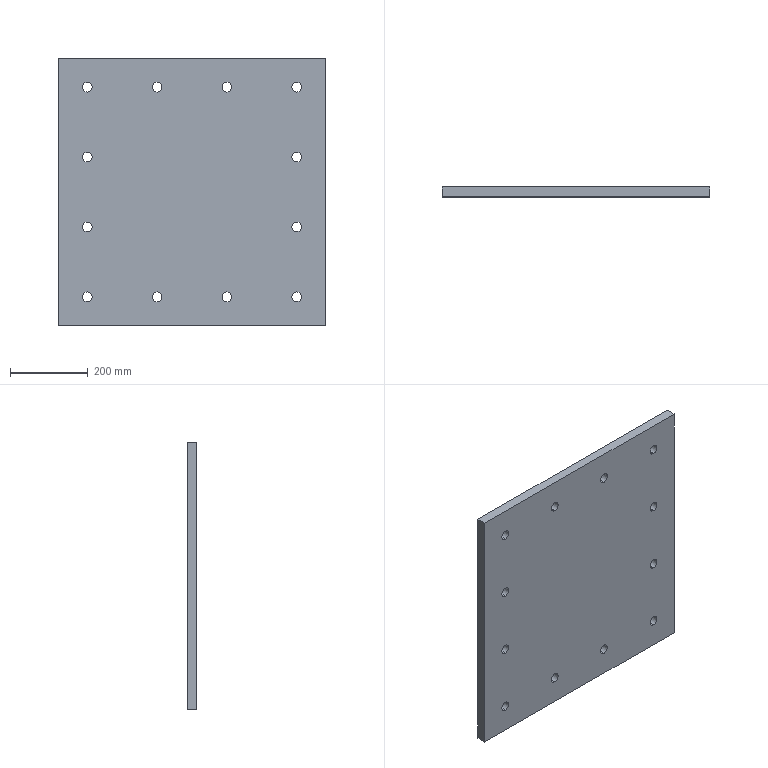Component | SolidWorks | Flange25-5 | 1 solid | 30 faces | box 690 x 25 x 690 mm | volume 11755238 mm3 | cylinder 24 | plane 6 | commonest cylinder face diameters 25 x24 | material Plain Carbon Steel
STEP:
#1=COLOUR_RGB('',0.7922,0.8196,0.9333);
#2=FILL_AREA_STYLE_COLOUR('',#1);
#3=FILL_AREA_STYLE('',(#2));
#4=SURFACE_STYLE_FILL_AREA(#3);
#5=SURFACE_SIDE_STYLE('',(#4));
#6=SURFACE_STYLE_USAGE(.BOTH.,#5);
#7=PRESENTATION_STYLE_ASSIGNMENT((#6));
#8=CARTESIAN_POINT('',(674.21,46.055,62.905));
#9=VERTEX_POINT('',#8);
#10=CARTESIAN_POINT('',(674.21,46.055,61.921));
#11=VERTEX_POINT('',#10);
#12=CARTESIAN_POINT('',(674.21,46.055,62.413));
#13=DIRECTION('',(0.,1.,-0.));
#14=DIRECTION('',(0.,0.,-1.));
#15=AXIS2_PLACEMENT_3D('',#12,#13,#14);
#16=CIRCLE('',#15,0.4921);
#17=EDGE_CURVE('',#9,#11,#16,.T.);
#18=ORIENTED_EDGE('',*,*,#17,.F.);
#19=CARTESIAN_POINT('',(674.21,47.039,62.905));
#20=VERTEX_POINT('',#19);
#21=CARTESIAN_POINT('',(674.21,46.055,62.905));
#22=DIRECTION('',(0.,1.,-0.));
#23=VECTOR('',#22,39.37);
#24=LINE('',#21,#23);
#25=EDGE_CURVE('',#9,#20,#24,.T.);
#26=ORIENTED_EDGE('',*,*,#25,.T.);
#27=CARTESIAN_POINT('',(674.21,47.039,61.921));
#28=VERTEX_POINT('',#27);
#29=CARTESIAN_POINT('',(674.21,47.039,62.413));
#30=DIRECTION('',(0.,1.,-0.));
#31=DIRECTION('',(0.,0.,-1.));
#32=AXIS2_PLACEMENT_3D('',#29,#30,#31);
#33=CIRCLE('',#32,0.4921);
#34=EDGE_CURVE('',#20,#28,#33,.T.);
#35=ORIENTED_EDGE('',*,*,#34,.T.);
#36=CARTESIAN_POINT('',(674.21,46.055,61.921));
#37=DIRECTION('',(0.,1.,-0.));
#38=VECTOR('',#37,39.37);
#39=LINE('',#36,#38);
#40=EDGE_CURVE('',#11,#28,#39,.T.);
#41=ORIENTED_EDGE('',*,*,#40,.F.);
#42=EDGE_LOOP('',(#18,#26,#35,#41));
#43=FACE_OUTER_BOUND('',#42,.T.);
#44=CARTESIAN_POINT('',(674.21,46.055,62.413));
#45=DIRECTION('',(0.,1.,-0.));
#46=DIRECTION('',(0.,0.,-1.));
#47=AXIS2_PLACEMENT_3D('',#44,#45,#46);
#48=CYLINDRICAL_SURFACE('',#47,0.4921);
#49=ADVANCED_FACE('',(#43),#48,.F.);
#50=CARTESIAN_POINT('',(674.21,46.055,69.992));
#51=VERTEX_POINT('',#50);
#52=CARTESIAN_POINT('',(674.21,46.055,69.007));
#53=VERTEX_POINT('',#52);
#54=CARTESIAN_POINT('',(674.21,46.055,69.499));
#55=DIRECTION('',(0.,1.,-0.));
#56=DIRECTION('',(0.,0.,-1.));
#57=AXIS2_PLACEMENT_3D('',#54,#55,#56);
#58=CIRCLE('',#57,0.4921);
#59=EDGE_CURVE('',#51,#53,#58,.T.);
#60=ORIENTED_EDGE('',*,*,#59,.F.);
#61=CARTESIAN_POINT('',(674.21,47.039,69.992));
#62=VERTEX_POINT('',#61);
#63=CARTESIAN_POINT('',(674.21,46.055,69.992));
#64=DIRECTION('',(0.,1.,-0.));
#65=VECTOR('',#64,39.37);
#66=LINE('',#63,#65);
#67=EDGE_CURVE('',#51,#62,#66,.T.);
#68=ORIENTED_EDGE('',*,*,#67,.T.);
#69=CARTESIAN_POINT('',(674.21,47.039,69.007));
#70=VERTEX_POINT('',#69);
#71=CARTESIAN_POINT('',(674.21,47.039,69.499));
#72=DIRECTION('',(0.,1.,-0.));
#73=DIRECTION('',(0.,0.,-1.));
#74=AXIS2_PLACEMENT_3D('',#71,#72,#73);
#75=CIRCLE('',#74,0.4921);
#76=EDGE_CURVE('',#62,#70,#75,.T.);
#77=ORIENTED_EDGE('',*,*,#76,.T.);
#78=CARTESIAN_POINT('',(674.21,46.055,69.007));
#79=DIRECTION('',(0.,1.,-0.));
#80=VECTOR('',#79,39.37);
#81=LINE('',#78,#80);
#82=EDGE_CURVE('',#53,#70,#81,.T.);
#83=ORIENTED_EDGE('',*,*,#82,.F.);
#84=EDGE_LOOP('',(#60,#68,#77,#83));
#85=FACE_OUTER_BOUND('',#84,.T.);
#86=CARTESIAN_POINT('',(674.21,46.055,69.499));
#87=DIRECTION('',(0.,1.,-0.));
#88=DIRECTION('',(0.,0.,-1.));
#89=AXIS2_PLACEMENT_3D('',#86,#87,#88);
#90=CYLINDRICAL_SURFACE('',#89,0.4921);
#91=ADVANCED_FACE('',(#85),#90,.F.);
#92=CARTESIAN_POINT('',(674.21,46.055,77.078));
#93=VERTEX_POINT('',#92);
#94=CARTESIAN_POINT('',(674.21,46.055,76.094));
#95=VERTEX_POINT('',#94);
#96=CARTESIAN_POINT('',(674.21,46.055,76.586));
#97=DIRECTION('',(0.,1.,-0.));
#98=DIRECTION('',(0.,0.,-1.));
#99=AXIS2_PLACEMENT_3D('',#96,#97,#98);
#100=CIRCLE('',#99,0.4921);
#101=EDGE_CURVE('',#93,#95,#100,.T.);
#102=ORIENTED_EDGE('',*,*,#101,.F.);
#103=CARTESIAN_POINT('',(674.21,47.039,77.078));
#104=VERTEX_POINT('',#103);
#105=CARTESIAN_POINT('',(674.21,46.055,77.078));
#106=DIRECTION('',(0.,1.,-0.));
#107=VECTOR('',#106,39.37);
#108=LINE('',#105,#107);
#109=EDGE_CURVE('',#93,#104,#108,.T.);
#110=ORIENTED_EDGE('',*,*,#109,.T.);
#111=CARTESIAN_POINT('',(674.21,47.039,76.094));
#112=VERTEX_POINT('',#111);
#113=CARTESIAN_POINT('',(674.21,47.039,76.586));
#114=DIRECTION('',(0.,1.,-0.));
#115=DIRECTION('',(0.,0.,-1.));
#116=AXIS2_PLACEMENT_3D('',#113,#114,#115);
#117=CIRCLE('',#116,0.4921);
#118=EDGE_CURVE('',#104,#112,#117,.T.);
#119=ORIENTED_EDGE('',*,*,#118,.T.);
#120=CARTESIAN_POINT('',(674.21,46.055,76.094));
#121=DIRECTION('',(0.,1.,-0.));
#122=VECTOR('',#121,39.37);
#123=LINE('',#120,#122);
#124=EDGE_CURVE('',#95,#112,#123,.T.);
#125=ORIENTED_EDGE('',*,*,#124,.F.);
#126=EDGE_LOOP('',(#102,#110,#119,#125));
#127=FACE_OUTER_BOUND('',#126,.T.);
#128=CARTESIAN_POINT('',(674.21,46.055,76.586));
#129=DIRECTION('',(0.,1.,-0.));
#130=DIRECTION('',(0.,0.,-1.));
#131=AXIS2_PLACEMENT_3D('',#128,#129,#130);
#132=CYLINDRICAL_SURFACE('',#131,0.4921);
#133=ADVANCED_FACE('',(#127),#132,.F.);
#134=CARTESIAN_POINT('',(652.95,46.055,62.905));
#135=VERTEX_POINT('',#134);
#136=CARTESIAN_POINT('',(652.95,46.055,61.921));
#137=VERTEX_POINT('',#136);
#138=CARTESIAN_POINT('',(652.95,46.055,62.413));
#139=DIRECTION('',(0.,1.,-0.));
#140=DIRECTION('',(0.,0.,-1.));
#141=AXIS2_PLACEMENT_3D('',#138,#139,#140);
#142=CIRCLE('',#141,0.4921);
#143=EDGE_CURVE('',#135,#137,#142,.T.);
#144=ORIENTED_EDGE('',*,*,#143,.F.);
#145=CARTESIAN_POINT('',(652.95,47.039,62.905));
#146=VERTEX_POINT('',#145);
#147=CARTESIAN_POINT('',(652.95,46.055,62.905));
#148=DIRECTION('',(0.,1.,-0.));
#149=VECTOR('',#148,39.37);
#150=LINE('',#147,#149);
#151=EDGE_CURVE('',#135,#146,#150,.T.);
#152=ORIENTED_EDGE('',*,*,#151,.T.);
#153=CARTESIAN_POINT('',(652.95,47.039,61.921));
#154=VERTEX_POINT('',#153);
#155=CARTESIAN_POINT('',(652.95,47.039,62.413));
#156=DIRECTION('',(0.,1.,-0.));
#157=DIRECTION('',(0.,0.,-1.));
#158=AXIS2_PLACEMENT_3D('',#155,#156,#157);
#159=CIRCLE('',#158,0.4921);
#160=EDGE_CURVE('',#146,#154,#159,.T.);
#161=ORIENTED_EDGE('',*,*,#160,.T.);
#162=CARTESIAN_POINT('',(652.95,46.055,61.921));
#163=DIRECTION('',(0.,1.,-0.));
#164=VECTOR('',#163,39.37);
#165=LINE('',#162,#164);
#166=EDGE_CURVE('',#137,#154,#165,.T.);
#167=ORIENTED_EDGE('',*,*,#166,.F.);
#168=EDGE_LOOP('',(#144,#152,#161,#167));
#169=FACE_OUTER_BOUND('',#168,.T.);
#170=CARTESIAN_POINT('',(652.95,46.055,62.413));
#171=DIRECTION('',(0.,1.,-0.));
#172=DIRECTION('',(0.,0.,-1.));
#173=AXIS2_PLACEMENT_3D('',#170,#171,#172);
#174=CYLINDRICAL_SURFACE('',#173,0.4921);
#175=ADVANCED_FACE('',(#169),#174,.F.);
#176=CARTESIAN_POINT('',(660.037,46.055,62.905));
#177=VERTEX_POINT('',#176);
#178=CARTESIAN_POINT('',(660.037,46.055,61.921));
#179=VERTEX_POINT('',#178);
#180=CARTESIAN_POINT('',(660.037,46.055,62.413));
#181=DIRECTION('',(0.,1.,-0.));
#182=DIRECTION('',(0.,0.,-1.));
#183=AXIS2_PLACEMENT_3D('',#180,#181,#182);
#184=CIRCLE('',#183,0.4921);
#185=EDGE_CURVE('',#177,#179,#184,.T.);
#186=ORIENTED_EDGE('',*,*,#185,.F.);
#187=CARTESIAN_POINT('',(660.037,47.039,62.905));
#188=VERTEX_POINT('',#187);
#189=CARTESIAN_POINT('',(660.037,46.055,62.905));
#190=DIRECTION('',(0.,1.,-0.));
#191=VECTOR('',#190,39.37);
#192=LINE('',#189,#191);
#193=EDGE_CURVE('',#177,#188,#192,.T.);
#194=ORIENTED_EDGE('',*,*,#193,.T.);
#195=CARTESIAN_POINT('',(660.037,47.039,61.921));
#196=VERTEX_POINT('',#195);
#197=CARTESIAN_POINT('',(660.037,47.039,62.413));
#198=DIRECTION('',(0.,1.,-0.));
#199=DIRECTION('',(0.,0.,-1.));
#200=AXIS2_PLACEMENT_3D('',#197,#198,#199);
#201=CIRCLE('',#200,0.4921);
#202=EDGE_CURVE('',#188,#196,#201,.T.);
#203=ORIENTED_EDGE('',*,*,#202,.T.);
#204=CARTESIAN_POINT('',(660.037,46.055,61.921));
#205=DIRECTION('',(0.,1.,-0.));
#206=VECTOR('',#205,39.37);
#207=LINE('',#204,#206);
#208=EDGE_CURVE('',#179,#196,#207,.T.);
#209=ORIENTED_EDGE('',*,*,#208,.F.);
#210=EDGE_LOOP('',(#186,#194,#203,#209));
#211=FACE_OUTER_BOUND('',#210,.T.);
#212=CARTESIAN_POINT('',(660.037,46.055,62.413));
#213=DIRECTION('',(0.,1.,-0.));
#214=DIRECTION('',(0.,0.,-1.));
#215=AXIS2_PLACEMENT_3D('',#212,#213,#214);
#216=CYLINDRICAL_SURFACE('',#215,0.4921);
#217=ADVANCED_FACE('',(#211),#216,.F.);
#218=CARTESIAN_POINT('',(667.124,46.055,62.905));
#219=VERTEX_POINT('',#218);
#220=CARTESIAN_POINT('',(667.124,46.055,61.921));
#221=VERTEX_POINT('',#220);
#222=CARTESIAN_POINT('',(667.124,46.055,62.413));
#223=DIRECTION('',(0.,1.,-0.));
#224=DIRECTION('',(0.,0.,-1.));
#225=AXIS2_PLACEMENT_3D('',#222,#223,#224);
#226=CIRCLE('',#225,0.4921);
#227=EDGE_CURVE('',#219,#221,#226,.T.);
#228=ORIENTED_EDGE('',*,*,#227,.F.);
#229=CARTESIAN_POINT('',(667.124,47.039,62.905));
#230=VERTEX_POINT('',#229);
#231=CARTESIAN_POINT('',(667.124,46.055,62.905));
#232=DIRECTION('',(0.,1.,-0.));
#233=VECTOR('',#232,39.37);
#234=LINE('',#231,#233);
#235=EDGE_CURVE('',#219,#230,#234,.T.);
#236=ORIENTED_EDGE('',*,*,#235,.T.);
#237=CARTESIAN_POINT('',(667.124,47.039,61.921));
#238=VERTEX_POINT('',#237);
#239=CARTESIAN_POINT('',(667.124,47.039,62.413));
#240=DIRECTION('',(0.,1.,-0.));
#241=DIRECTION('',(0.,0.,-1.));
#242=AXIS2_PLACEMENT_3D('',#239,#240,#241);
#243=CIRCLE('',#242,0.4921);
#244=EDGE_CURVE('',#230,#238,#243,.T.);
#245=ORIENTED_EDGE('',*,*,#244,.T.);
#246=CARTESIAN_POINT('',(667.124,46.055,61.921));
#247=DIRECTION('',(0.,1.,-0.));
#248=VECTOR('',#247,39.37);
#249=LINE('',#246,#248);
#250=EDGE_CURVE('',#221,#238,#249,.T.);
#251=ORIENTED_EDGE('',*,*,#250,.F.);
#252=EDGE_LOOP('',(#228,#236,#245,#251));
#253=FACE_OUTER_BOUND('',#252,.T.);
#254=CARTESIAN_POINT('',(667.124,46.055,62.413));
#255=DIRECTION('',(0.,1.,-0.));
#256=DIRECTION('',(0.,0.,-1.));
#257=AXIS2_PLACEMENT_3D('',#254,#255,#256);
#258=CYLINDRICAL_SURFACE('',#257,0.4921);
#259=ADVANCED_FACE('',(#253),#258,.F.);
#260=CARTESIAN_POINT('',(652.95,46.055,69.992));
#261=VERTEX_POINT('',#260);
#262=CARTESIAN_POINT('',(652.95,46.055,69.007));
#263=VERTEX_POINT('',#262);
#264=CARTESIAN_POINT('',(652.95,46.055,69.499));
#265=DIRECTION('',(0.,1.,-0.));
#266=DIRECTION('',(0.,0.,-1.));
#267=AXIS2_PLACEMENT_3D('',#264,#265,#266);
#268=CIRCLE('',#267,0.4921);
#269=EDGE_CURVE('',#261,#263,#268,.T.);
#270=ORIENTED_EDGE('',*,*,#269,.F.);
#271=CARTESIAN_POINT('',(652.95,47.039,69.992));
#272=VERTEX_POINT('',#271);
#273=CARTESIAN_POINT('',(652.95,46.055,69.992));
#274=DIRECTION('',(0.,1.,-0.));
#275=VECTOR('',#274,39.37);
#276=LINE('',#273,#275);
#277=EDGE_CURVE('',#261,#272,#276,.T.);
#278=ORIENTED_EDGE('',*,*,#277,.T.);
#279=CARTESIAN_POINT('',(652.95,47.039,69.007));
#280=VERTEX_POINT('',#279);
#281=CARTESIAN_POINT('',(652.95,47.039,69.499));
#282=DIRECTION('',(0.,1.,-0.));
#283=DIRECTION('',(0.,0.,-1.));
#284=AXIS2_PLACEMENT_3D('',#281,#282,#283);
#285=CIRCLE('',#284,0.4921);
#286=EDGE_CURVE('',#272,#280,#285,.T.);
#287=ORIENTED_EDGE('',*,*,#286,.T.);
#288=CARTESIAN_POINT('',(652.95,46.055,69.007));
#289=DIRECTION('',(0.,1.,-0.));
#290=VECTOR('',#289,39.37);
#291=LINE('',#288,#290);
#292=EDGE_CURVE('',#263,#280,#291,.T.);
#293=ORIENTED_EDGE('',*,*,#292,.F.);
#294=EDGE_LOOP('',(#270,#278,#287,#293));
#295=FACE_OUTER_BOUND('',#294,.T.);
#296=CARTESIAN_POINT('',(652.95,46.055,69.499));
#297=DIRECTION('',(0.,1.,-0.));
#298=DIRECTION('',(0.,0.,-1.));
#299=AXIS2_PLACEMENT_3D('',#296,#297,#298);
#300=CYLINDRICAL_SURFACE('',#299,0.4921);
#301=ADVANCED_FACE('',(#295),#300,.F.);
#302=CARTESIAN_POINT('',(652.95,46.055,77.078));
#303=VERTEX_POINT('',#302);
#304=CARTESIAN_POINT('',(652.95,46.055,76.094));
#305=VERTEX_POINT('',#304);
#306=CARTESIAN_POINT('',(652.95,46.055,76.586));
#307=DIRECTION('',(0.,1.,-0.));
#308=DIRECTION('',(0.,0.,-1.));
#309=AXIS2_PLACEMENT_3D('',#306,#307,#308);
#310=CIRCLE('',#309,0.4921);
#311=EDGE_CURVE('',#303,#305,#310,.T.);
#312=ORIENTED_EDGE('',*,*,#311,.F.);
#313=CARTESIAN_POINT('',(652.95,47.039,77.078));
#314=VERTEX_POINT('',#313);
#315=CARTESIAN_POINT('',(652.95,46.055,77.078));
#316=DIRECTION('',(0.,1.,-0.));
#317=VECTOR('',#316,39.37);
#318=LINE('',#315,#317);
#319=EDGE_CURVE('',#303,#314,#318,.T.);
#320=ORIENTED_EDGE('',*,*,#319,.T.);
#321=CARTESIAN_POINT('',(652.95,47.039,76.094));
#322=VERTEX_POINT('',#321);
#323=CARTESIAN_POINT('',(652.95,47.039,76.586));
#324=DIRECTION('',(0.,1.,-0.));
#325=DIRECTION('',(0.,0.,-1.));
#326=AXIS2_PLACEMENT_3D('',#323,#324,#325);
#327=CIRCLE('',#326,0.4921);
#328=EDGE_CURVE('',#314,#322,#327,.T.);
#329=ORIENTED_EDGE('',*,*,#328,.T.);
#330=CARTESIAN_POINT('',(652.95,46.055,76.094));
#331=DIRECTION('',(0.,1.,-0.));
#332=VECTOR('',#331,39.37);
#333=LINE('',#330,#332);
#334=EDGE_CURVE('',#305,#322,#333,.T.);
#335=ORIENTED_EDGE('',*,*,#334,.F.);
#336=EDGE_LOOP('',(#312,#320,#329,#335));
#337=FACE_OUTER_BOUND('',#336,.T.);
#338=CARTESIAN_POINT('',(652.95,46.055,76.586));
#339=DIRECTION('',(0.,1.,-0.));
#340=DIRECTION('',(0.,0.,-1.));
#341=AXIS2_PLACEMENT_3D('',#338,#339,#340);
#342=CYLINDRICAL_SURFACE('',#341,0.4921);
#343=ADVANCED_FACE('',(#337),#342,.F.);
#344=CARTESIAN_POINT('',(652.95,46.055,84.165));
#345=VERTEX_POINT('',#344);
#346=CARTESIAN_POINT('',(652.95,46.055,83.181));
#347=VERTEX_POINT('',#346);
#348=CARTESIAN_POINT('',(652.95,46.055,83.673));
#349=DIRECTION('',(0.,1.,-0.));
#350=DIRECTION('',(0.,0.,-1.));
#351=AXIS2_PLACEMENT_3D('',#348,#349,#350);
#352=CIRCLE('',#351,0.4921);
#353=EDGE_CURVE('',#345,#347,#352,.T.);
#354=ORIENTED_EDGE('',*,*,#353,.F.);
#355=CARTESIAN_POINT('',(652.95,47.039,84.165));
#356=VERTEX_POINT('',#355);
#357=CARTESIAN_POINT('',(652.95,46.055,84.165));
#358=DIRECTION('',(0.,1.,-0.));
#359=VECTOR('',#358,39.37);
#360=LINE('',#357,#359);
#361=EDGE_CURVE('',#345,#356,#360,.T.);
#362=ORIENTED_EDGE('',*,*,#361,.T.);
#363=CARTESIAN_POINT('',(652.95,47.039,83.181));
#364=VERTEX_POINT('',#363);
#365=CARTESIAN_POINT('',(652.95,47.039,83.673));
#366=DIRECTION('',(0.,1.,-0.));
#367=DIRECTION('',(0.,0.,-1.));
#368=AXIS2_PLACEMENT_3D('',#365,#366,#367);
#369=CIRCLE('',#368,0.4921);
#370=EDGE_CURVE('',#356,#364,#369,.T.);
#371=ORIENTED_EDGE('',*,*,#370,.T.);
#372=CARTESIAN_POINT('',(652.95,46.055,83.181));
#373=DIRECTION('',(0.,1.,-0.));
#374=VECTOR('',#373,39.37);
#375=LINE('',#372,#374);
#376=EDGE_CURVE('',#347,#364,#375,.T.);
#377=ORIENTED_EDGE('',*,*,#376,.F.);
#378=EDGE_LOOP('',(#354,#362,#371,#377));
#379=FACE_OUTER_BOUND('',#378,.T.);
#380=CARTESIAN_POINT('',(652.95,46.055,83.673));
#381=DIRECTION('',(0.,1.,-0.));
#382=DIRECTION('',(0.,0.,-1.));
#383=AXIS2_PLACEMENT_3D('',#380,#381,#382);
#384=CYLINDRICAL_SURFACE('',#383,0.4921);
#385=ADVANCED_FACE('',(#379),#384,.F.);
#386=CARTESIAN_POINT('',(660.037,46.055,84.165));
#387=VERTEX_POINT('',#386);
#388=CARTESIAN_POINT('',(660.037,46.055,83.181));
#389=VERTEX_POINT('',#388);
#390=CARTESIAN_POINT('',(660.037,46.055,83.673));
#391=DIRECTION('',(0.,1.,-0.));
#392=DIRECTION('',(0.,0.,-1.));
#393=AXIS2_PLACEMENT_3D('',#390,#391,#392);
#394=CIRCLE('',#393,0.4921);
#395=EDGE_CURVE('',#387,#389,#394,.T.);
#396=ORIENTED_EDGE('',*,*,#395,.F.);
#397=CARTESIAN_POINT('',(660.037,47.039,84.165));
#398=VERTEX_POINT('',#397);
#399=CARTESIAN_POINT('',(660.037,46.055,84.165));
#400=DIRECTION('',(0.,1.,-0.));
#401=VECTOR('',#400,39.37);
#402=LINE('',#399,#401);
#403=EDGE_CURVE('',#387,#398,#402,.T.);
#404=ORIENTED_EDGE('',*,*,#403,.T.);
#405=CARTESIAN_POINT('',(660.037,47.039,83.181));
#406=VERTEX_POINT('',#405);
#407=CARTESIAN_POINT('',(660.037,47.039,83.673));
#408=DIRECTION('',(0.,1.,-0.));
#409=DIRECTION('',(0.,0.,-1.));
#410=AXIS2_PLACEMENT_3D('',#407,#408,#409);
#411=CIRCLE('',#410,0.4921);
#412=EDGE_CURVE('',#398,#406,#411,.T.);
#413=ORIENTED_EDGE('',*,*,#412,.T.);
#414=CARTESIAN_POINT('',(660.037,46.055,83.181));
#415=DIRECTION('',(0.,1.,-0.));
#416=VECTOR('',#415,39.37);
#417=LINE('',#414,#416);
#418=EDGE_CURVE('',#389,#406,#417,.T.);
#419=ORIENTED_EDGE('',*,*,#418,.F.);
#420=EDGE_LOOP('',(#396,#404,#413,#419));
#421=FACE_OUTER_BOUND('',#420,.T.);
#422=CARTESIAN_POINT('',(660.037,46.055,83.673));
#423=DIRECTION('',(0.,1.,-0.));
#424=DIRECTION('',(0.,0.,-1.));
#425=AXIS2_PLACEMENT_3D('',#422,#423,#424);
#426=CYLINDRICAL_SURFACE('',#425,0.4921);
#427=ADVANCED_FACE('',(#421),#426,.F.);
#428=CARTESIAN_POINT('',(667.124,46.055,84.165));
#429=VERTEX_POINT('',#428);
#430=CARTESIAN_POINT('',(667.124,46.055,83.181));
#431=VERTEX_POINT('',#430);
#432=CARTESIAN_POINT('',(667.124,46.055,83.673));
#433=DIRECTION('',(0.,1.,-0.));
#434=DIRECTION('',(0.,0.,-1.));
#435=AXIS2_PLACEMENT_3D('',#432,#433,#434);
#436=CIRCLE('',#435,0.4921);
#437=EDGE_CURVE('',#429,#431,#436,.T.);
#438=ORIENTED_EDGE('',*,*,#437,.F.);
#439=CARTESIAN_POINT('',(667.124,47.039,84.165));
#440=VERTEX_POINT('',#439);
#441=CARTESIAN_POINT('',(667.124,46.055,84.165));
#442=DIRECTION('',(0.,1.,-0.));
#443=VECTOR('',#442,39.37);
#444=LINE('',#441,#443);
#445=EDGE_CURVE('',#429,#440,#444,.T.);
#446=ORIENTED_EDGE('',*,*,#445,.T.);
#447=CARTESIAN_POINT('',(667.124,47.039,83.181));
#448=VERTEX_POINT('',#447);
#449=CARTESIAN_POINT('',(667.124,47.039,83.673));
#450=DIRECTION('',(0.,1.,-0.));
#451=DIRECTION('',(0.,0.,-1.));
#452=AXIS2_PLACEMENT_3D('',#449,#450,#451);
#453=CIRCLE('',#452,0.4921);
#454=EDGE_CURVE('',#440,#448,#453,.T.);
#455=ORIENTED_EDGE('',*,*,#454,.T.);
#456=CARTESIAN_POINT('',(667.124,46.055,83.181));
#457=DIRECTION('',(0.,1.,-0.));
#458=VECTOR('',#457,39.37);
#459=LINE('',#456,#458);
#460=EDGE_CURVE('',#431,#448,#459,.T.);
#461=ORIENTED_EDGE('',*,*,#460,.F.);
#462=EDGE_LOOP('',(#438,#446,#455,#461));
#463=FACE_OUTER_BOUND('',#462,.T.);
#464=CARTESIAN_POINT('',(667.124,46.055,83.673));
#465=DIRECTION('',(0.,1.,-0.));
#466=DIRECTION('',(0.,0.,-1.));
#467=AXIS2_PLACEMENT_3D('',#464,#465,#466);
#468=CYLINDRICAL_SURFACE('',#467,0.4921);
#469=ADVANCED_FACE('',(#463),#468,.F.);
#470=CARTESIAN_POINT('',(674.21,46.055,84.165));
#471=VERTEX_POINT('',#470);
#472=CARTESIAN_POINT('',(674.21,46.055,83.181));
#473=VERTEX_POINT('',#472);
#474=CARTESIAN_POINT('',(674.21,46.055,83.673));
#475=DIRECTION('',(0.,1.,-0.));
#476=DIRECTION('',(0.,0.,-1.));
#477=AXIS2_PLACEMENT_3D('',#474,#475,#476);
#478=CIRCLE('',#477,0.4921);
#479=EDGE_CURVE('',#471,#473,#478,.T.);
#480=ORIENTED_EDGE('',*,*,#479,.F.);
#481=CARTESIAN_POINT('',(674.21,47.039,84.165));
#482=VERTEX_POINT('',#481);
#483=CARTESIAN_POINT('',(674.21,46.055,84.165));
#484=DIRECTION('',(0.,1.,-0.));
#485=VECTOR('',#484,39.37);
#486=LINE('',#483,#485);
#487=EDGE_CURVE('',#471,#482,#486,.T.);
#488=ORIENTED_EDGE('',*,*,#487,.T.);
#489=CARTESIAN_POINT('',(674.21,47.039,83.181));
#490=VERTEX_POINT('',#489);
#491=CARTESIAN_POINT('',(674.21,47.039,83.673));
#492=DIRECTION('',(0.,1.,-0.));
#493=DIRECTION('',(0.,0.,-1.));
#494=AXIS2_PLACEMENT_3D('',#491,#492,#493);
#495=CIRCLE('',#494,0.4921);
#496=EDGE_CURVE('',#482,#490,#495,.T.);
#497=ORIENTED_EDGE('',*,*,#496,.T.);
#498=CARTESIAN_POINT('',(674.21,46.055,83.181));
#499=DIRECTION('',(0.,1.,-0.));
#500=VECTOR('',#499,39.37);
#501=LINE('',#498,#500);
#502=EDGE_CURVE('',#473,#490,#501,.T.);
#503=ORIENTED_EDGE('',*,*,#502,.F.);
#504=EDGE_LOOP('',(#480,#488,#497,#503));
#505=FACE_OUTER_BOUND('',#504,.T.);
#506=CARTESIAN_POINT('',(674.21,46.055,83.673));
#507=DIRECTION('',(0.,1.,-0.));
#508=DIRECTION('',(0.,0.,-1.));
#509=AXIS2_PLACEMENT_3D('',#506,#507,#508);
#510=CYLINDRICAL_SURFACE('',#509,0.4921);
#511=ADVANCED_FACE('',(#505),#510,.F.);
#512=CARTESIAN_POINT('',(649.998,47.039,59.46));
#513=VERTEX_POINT('',#512);
#514=CARTESIAN_POINT('',(649.998,47.039,86.625));
#515=VERTEX_POINT('',#514);
#516=CARTESIAN_POINT('',(649.998,47.039,86.625));
#517=DIRECTION('',(0.,-0.,1.));
#518=VECTOR('',#517,39.37);
#519=LINE('',#516,#518);
#520=EDGE_CURVE('',#513,#515,#519,.T.);
#521=ORIENTED_EDGE('',*,*,#520,.F.);
#522=CARTESIAN_POINT('',(649.998,46.055,59.46));
#523=VERTEX_POINT('',#522);
#524=CARTESIAN_POINT('',(649.998,46.055,59.46));
#525=DIRECTION('',(0.,1.,-0.));
#526=VECTOR('',#525,39.37);
#527=LINE('',#524,#526);
#528=EDGE_CURVE('',#523,#513,#527,.T.);
#529=ORIENTED_EDGE('',*,*,#528,.F.);
#530=CARTESIAN_POINT('',(649.998,46.055,86.625));
#531=VERTEX_POINT('',#530);
#532=CARTESIAN_POINT('',(649.998,46.055,86.625));
#533=DIRECTION('',(0.,-0.,1.));
#534=VECTOR('',#533,39.37);
#535=LINE('',#532,#534);
#536=EDGE_CURVE('',#523,#531,#535,.T.);
#537=ORIENTED_EDGE('',*,*,#536,.T.);
#538=CARTESIAN_POINT('',(649.998,46.055,86.625));
#539=DIRECTION('',(0.,1.,-0.));
#540=VECTOR('',#539,39.37);
#541=LINE('',#538,#540);
#542=EDGE_CURVE('',#531,#515,#541,.T.);
#543=ORIENTED_EDGE('',*,*,#542,.T.);
#544=EDGE_LOOP('',(#521,#529,#537,#543));
#545=FACE_OUTER_BOUND('',#544,.T.);
#546=CARTESIAN_POINT('',(649.998,46.055,86.625));
#547=DIRECTION('',(-1.,0.,0.));
#548=DIRECTION('',(0.,-0.,1.));
#549=AXIS2_PLACEMENT_3D('',#546,#547,#548);
#550=PLANE('',#549);
#551=ADVANCED_FACE('',(#545),#550,.T.);
#552=CARTESIAN_POINT('',(677.163,47.039,59.46));
#553=VERTEX_POINT('',#552);
#554=CARTESIAN_POINT('',(677.163,47.039,59.46));
#555=DIRECTION('',(-1.,0.,0.));
#556=VECTOR('',#555,39.37);
#557=LINE('',#554,#556);
#558=EDGE_CURVE('',#553,#513,#557,.T.);
#559=ORIENTED_EDGE('',*,*,#558,.F.);
#560=CARTESIAN_POINT('',(677.163,46.055,59.46));
#561=VERTEX_POINT('',#560);
#562=CARTESIAN_POINT('',(677.163,46.055,59.46));
#563=DIRECTION('',(0.,1.,-0.));
#564=VECTOR('',#563,39.37);
#565=LINE('',#562,#564);
#566=EDGE_CURVE('',#561,#553,#565,.T.);
#567=ORIENTED_EDGE('',*,*,#566,.F.);
#568=CARTESIAN_POINT('',(677.163,46.055,59.46));
#569=DIRECTION('',(-1.,0.,0.));
#570=VECTOR('',#569,39.37);
#571=LINE('',#568,#570);
#572=EDGE_CURVE('',#561,#523,#571,.T.);
#573=ORIENTED_EDGE('',*,*,#572,.T.);
#574=ORIENTED_EDGE('',*,*,#528,.T.);
#575=EDGE_LOOP('',(#559,#567,#573,#574));
#576=FACE_OUTER_BOUND('',#575,.T.);
#577=CARTESIAN_POINT('',(677.163,46.055,59.46));
#578=DIRECTION('',(-0.,0.,-1.));
#579=DIRECTION('',(-1.,0.,0.));
#580=AXIS2_PLACEMENT_3D('',#577,#578,#579);
#581=PLANE('',#580);
#582=ADVANCED_FACE('',(#576),#581,.T.);
#583=CARTESIAN_POINT('',(677.163,47.039,86.625));
#584=VERTEX_POINT('',#583);
#585=CARTESIAN_POINT('',(677.163,47.039,86.625));
#586=DIRECTION('',(-0.,0.,-1.));
#587=VECTOR('',#586,39.37);
#588=LINE('',#585,#587);
#589=EDGE_CURVE('',#584,#553,#588,.T.);
#590=ORIENTED_EDGE('',*,*,#589,.F.);
#591=CARTESIAN_POINT('',(677.163,46.055,86.625));
#592=VERTEX_POINT('',#591);
#593=CARTESIAN_POINT('',(677.163,46.055,86.625));
#594=DIRECTION('',(0.,1.,-0.));
#595=VECTOR('',#594,39.37);
#596=LINE('',#593,#595);
#597=EDGE_CURVE('',#592,#584,#596,.T.);
#598=ORIENTED_EDGE('',*,*,#597,.F.);
#599=CARTESIAN_POINT('',(677.163,46.055,86.625));
#600=DIRECTION('',(-0.,0.,-1.));
#601=VECTOR('',#600,39.37);
#602=LINE('',#599,#601);
#603=EDGE_CURVE('',#592,#561,#602,.T.);
#604=ORIENTED_EDGE('',*,*,#603,.T.);
#605=ORIENTED_EDGE('',*,*,#566,.T.);
#606=EDGE_LOOP('',(#590,#598,#604,#605));
#607=FACE_OUTER_BOUND('',#606,.T.);
#608=CARTESIAN_POINT('',(677.163,46.055,86.625));
#609=DIRECTION('',(1.,-0.,-0.));
#610=DIRECTION('',(-0.,0.,-1.));
#611=AXIS2_PLACEMENT_3D('',#608,#609,#610);
#612=PLANE('',#611);
#613=ADVANCED_FACE('',(#607),#612,.T.);
#614=CARTESIAN_POINT('',(677.163,47.039,86.625));
#615=DIRECTION('',(1.,-0.,-0.));
#616=VECTOR('',#615,39.37);
#617=LINE('',#614,#616);
#618=EDGE_CURVE('',#515,#584,#617,.T.);
#619=ORIENTED_EDGE('',*,*,#618,.F.);
#620=ORIENTED_EDGE('',*,*,#542,.F.);
#621=CARTESIAN_POINT('',(677.163,46.055,86.625));
#622=DIRECTION('',(1.,-0.,-0.));
#623=VECTOR('',#622,39.37);
#624=LINE('',#621,#623);
#625=EDGE_CURVE('',#531,#592,#624,.T.);
#626=ORIENTED_EDGE('',*,*,#625,.T.);
#627=ORIENTED_EDGE('',*,*,#597,.T.);
#628=EDGE_LOOP('',(#619,#620,#626,#627));
#629=FACE_OUTER_BOUND('',#628,.T.);
#630=CARTESIAN_POINT('',(677.163,46.055,86.625));
#631=DIRECTION('',(0.,-0.,1.));
#632=DIRECTION('',(1.,-0.,-0.));
#633=AXIS2_PLACEMENT_3D('',#630,#631,#632);
#634=PLANE('',#633);
#635=ADVANCED_FACE('',(#629),#634,.T.);
#636=CARTESIAN_POINT('',(674.21,46.055,62.413));
#637=DIRECTION('',(0.,1.,-0.));
#638=DIRECTION('',(0.,0.,-1.));
#639=AXIS2_PLACEMENT_3D('',#636,#637,#638);
#640=CIRCLE('',#639,0.4921);
#641=EDGE_CURVE('',#11,#9,#640,.T.);
#642=ORIENTED_EDGE('',*,*,#641,.T.);
#643=ORIENTED_EDGE('',*,*,#17,.T.);
#644=EDGE_LOOP('',(#642,#643));
#645=FACE_BOUND('',#644,.T.);
#646=CARTESIAN_POINT('',(674.21,46.055,69.499));
#647=DIRECTION('',(0.,1.,-0.));
#648=DIRECTION('',(0.,0.,-1.));
#649=AXIS2_PLACEMENT_3D('',#646,#647,#648);
#650=CIRCLE('',#649,0.4921);
#651=EDGE_CURVE('',#53,#51,#650,.T.);
#652=ORIENTED_EDGE('',*,*,#651,.T.);
#653=ORIENTED_EDGE('',*,*,#59,.T.);
#654=EDGE_LOOP('',(#652,#653));
#655=FACE_BOUND('',#654,.T.);
#656=CARTESIAN_POINT('',(674.21,46.055,76.586));
#657=DIRECTION('',(0.,1.,-0.));
#658=DIRECTION('',(0.,0.,-1.));
#659=AXIS2_PLACEMENT_3D('',#656,#657,#658);
#660=CIRCLE('',#659,0.4921);
#661=EDGE_CURVE('',#95,#93,#660,.T.);
#662=ORIENTED_EDGE('',*,*,#661,.T.);
#663=ORIENTED_EDGE('',*,*,#101,.T.);
#664=EDGE_LOOP('',(#662,#663));
#665=FACE_BOUND('',#664,.T.);
#666=CARTESIAN_POINT('',(652.95,46.055,62.413));
#667=DIRECTION('',(0.,1.,-0.));
#668=DIRECTION('',(0.,0.,-1.));
#669=AXIS2_PLACEMENT_3D('',#666,#667,#668);
#670=CIRCLE('',#669,0.4921);
#671=EDGE_CURVE('',#137,#135,#670,.T.);
#672=ORIENTED_EDGE('',*,*,#671,.T.);
#673=ORIENTED_EDGE('',*,*,#143,.T.);
#674=EDGE_LOOP('',(#672,#673));
#675=FACE_BOUND('',#674,.T.);
#676=CARTESIAN_POINT('',(660.037,46.055,62.413));
#677=DIRECTION('',(0.,1.,-0.));
#678=DIRECTION('',(0.,0.,-1.));
#679=AXIS2_PLACEMENT_3D('',#676,#677,#678);
#680=CIRCLE('',#679,0.4921);
#681=EDGE_CURVE('',#179,#177,#680,.T.);
#682=ORIENTED_EDGE('',*,*,#681,.T.);
#683=ORIENTED_EDGE('',*,*,#185,.T.);
#684=EDGE_LOOP('',(#682,#683));
#685=FACE_BOUND('',#684,.T.);
#686=CARTESIAN_POINT('',(667.124,46.055,62.413));
#687=DIRECTION('',(0.,1.,-0.));
#688=DIRECTION('',(0.,0.,-1.));
#689=AXIS2_PLACEMENT_3D('',#686,#687,#688);
#690=CIRCLE('',#689,0.4921);
#691=EDGE_CURVE('',#221,#219,#690,.T.);
#692=ORIENTED_EDGE('',*,*,#691,.T.);
#693=ORIENTED_EDGE('',*,*,#227,.T.);
#694=EDGE_LOOP('',(#692,#693));
#695=FACE_BOUND('',#694,.T.);
#696=CARTESIAN_POINT('',(652.95,46.055,69.499));
#697=DIRECTION('',(0.,1.,-0.));
#698=DIRECTION('',(0.,0.,-1.));
#699=AXIS2_PLACEMENT_3D('',#696,#697,#698);
#700=CIRCLE('',#699,0.4921);
#701=EDGE_CURVE('',#263,#261,#700,.T.);
#702=ORIENTED_EDGE('',*,*,#701,.T.);
#703=ORIENTED_EDGE('',*,*,#269,.T.);
#704=EDGE_LOOP('',(#702,#703));
#705=FACE_BOUND('',#704,.T.);
#706=CARTESIAN_POINT('',(652.95,46.055,76.586));
#707=DIRECTION('',(0.,1.,-0.));
#708=DIRECTION('',(0.,0.,-1.));
#709=AXIS2_PLACEMENT_3D('',#706,#707,#708);
#710=CIRCLE('',#709,0.4921);
#711=EDGE_CURVE('',#305,#303,#710,.T.);
#712=ORIENTED_EDGE('',*,*,#711,.T.);
#713=ORIENTED_EDGE('',*,*,#311,.T.);
#714=EDGE_LOOP('',(#712,#713));
#715=FACE_BOUND('',#714,.T.);
#716=CARTESIAN_POINT('',(652.95,46.055,83.673));
#717=DIRECTION('',(0.,1.,-0.));
#718=DIRECTION('',(0.,0.,-1.));
#719=AXIS2_PLACEMENT_3D('',#716,#717,#718);
#720=CIRCLE('',#719,0.4921);
#721=EDGE_CURVE('',#347,#345,#720,.T.);
#722=ORIENTED_EDGE('',*,*,#721,.T.);
#723=ORIENTED_EDGE('',*,*,#353,.T.);
#724=EDGE_LOOP('',(#722,#723));
#725=FACE_BOUND('',#724,.T.);
#726=CARTESIAN_POINT('',(660.037,46.055,83.673));
#727=DIRECTION('',(0.,1.,-0.));
#728=DIRECTION('',(0.,0.,-1.));
#729=AXIS2_PLACEMENT_3D('',#726,#727,#728);
#730=CIRCLE('',#729,0.4921);
#731=EDGE_CURVE('',#389,#387,#730,.T.);
#732=ORIENTED_EDGE('',*,*,#731,.T.);
#733=ORIENTED_EDGE('',*,*,#395,.T.);
#734=EDGE_LOOP('',(#732,#733));
#735=FACE_BOUND('',#734,.T.);
#736=CARTESIAN_POINT('',(667.124,46.055,83.673));
#737=DIRECTION('',(0.,1.,-0.));
#738=DIRECTION('',(0.,0.,-1.));
#739=AXIS2_PLACEMENT_3D('',#736,#737,#738);
#740=CIRCLE('',#739,0.4921);
#741=EDGE_CURVE('',#431,#429,#740,.T.);
#742=ORIENTED_EDGE('',*,*,#741,.T.);
#743=ORIENTED_EDGE('',*,*,#437,.T.);
#744=EDGE_LOOP('',(#742,#743));
#745=FACE_BOUND('',#744,.T.);
#746=CARTESIAN_POINT('',(674.21,46.055,83.673));
#747=DIRECTION('',(0.,1.,-0.));
#748=DIRECTION('',(0.,0.,-1.));
#749=AXIS2_PLACEMENT_3D('',#746,#747,#748);
#750=CIRCLE('',#749,0.4921);
#751=EDGE_CURVE('',#473,#471,#750,.T.);
#752=ORIENTED_EDGE('',*,*,#751,.T.);
#753=ORIENTED_EDGE('',*,*,#479,.T.);
#754=EDGE_LOOP('',(#752,#753));
#755=FACE_BOUND('',#754,.T.);
#756=ORIENTED_EDGE('',*,*,#536,.F.);
#757=ORIENTED_EDGE('',*,*,#572,.F.);
#758=ORIENTED_EDGE('',*,*,#603,.F.);
#759=ORIENTED_EDGE('',*,*,#625,.F.);
#760=EDGE_LOOP('',(#756,#757,#758,#759));
#761=FACE_OUTER_BOUND('',#760,.T.);
#762=CARTESIAN_POINT('',(663.58,46.055,73.043));
#763=DIRECTION('',(0.,1.,-0.));
#764=DIRECTION('',(-0.,0.,-1.));
#765=AXIS2_PLACEMENT_3D('',#762,#763,#764);
#766=PLANE('',#765);
#767=ADVANCED_FACE('',(#645,#655,#665,#675,#685,#695,#705,#715,#725,#735,#745,#755,#761),#766,.F.);
#768=CARTESIAN_POINT('',(674.21,47.039,62.413));
#769=DIRECTION('',(0.,1.,-0.));
#770=DIRECTION('',(0.,0.,-1.));
#771=AXIS2_PLACEMENT_3D('',#768,#769,#770);
#772=CIRCLE('',#771,0.4921);
#773=EDGE_CURVE('',#28,#20,#772,.T.);
#774=ORIENTED_EDGE('',*,*,#773,.F.);
#775=ORIENTED_EDGE('',*,*,#34,.F.);
#776=EDGE_LOOP('',(#774,#775));
#777=FACE_BOUND('',#776,.T.);
#778=CARTESIAN_POINT('',(674.21,47.039,69.499));
#779=DIRECTION('',(0.,1.,-0.));
#780=DIRECTION('',(0.,0.,-1.));
#781=AXIS2_PLACEMENT_3D('',#778,#779,#780);
#782=CIRCLE('',#781,0.4921);
#783=EDGE_CURVE('',#70,#62,#782,.T.);
#784=ORIENTED_EDGE('',*,*,#783,.F.);
#785=ORIENTED_EDGE('',*,*,#76,.F.);
#786=EDGE_LOOP('',(#784,#785));
#787=FACE_BOUND('',#786,.T.);
#788=CARTESIAN_POINT('',(674.21,47.039,76.586));
#789=DIRECTION('',(0.,1.,-0.));
#790=DIRECTION('',(0.,0.,-1.));
#791=AXIS2_PLACEMENT_3D('',#788,#789,#790);
#792=CIRCLE('',#791,0.4921);
#793=EDGE_CURVE('',#112,#104,#792,.T.);
#794=ORIENTED_EDGE('',*,*,#793,.F.);
#795=ORIENTED_EDGE('',*,*,#118,.F.);
#796=EDGE_LOOP('',(#794,#795));
#797=FACE_BOUND('',#796,.T.);
#798=CARTESIAN_POINT('',(652.95,47.039,62.413));
#799=DIRECTION('',(0.,1.,-0.));
#800=DIRECTION('',(0.,0.,-1.));
#801=AXIS2_PLACEMENT_3D('',#798,#799,#800);
#802=CIRCLE('',#801,0.4921);
#803=EDGE_CURVE('',#154,#146,#802,.T.);
#804=ORIENTED_EDGE('',*,*,#803,.F.);
#805=ORIENTED_EDGE('',*,*,#160,.F.);
#806=EDGE_LOOP('',(#804,#805));
#807=FACE_BOUND('',#806,.T.);
#808=CARTESIAN_POINT('',(660.037,47.039,62.413));
#809=DIRECTION('',(0.,1.,-0.));
#810=DIRECTION('',(0.,0.,-1.));
#811=AXIS2_PLACEMENT_3D('',#808,#809,#810);
#812=CIRCLE('',#811,0.4921);
#813=EDGE_CURVE('',#196,#188,#812,.T.);
#814=ORIENTED_EDGE('',*,*,#813,.F.);
#815=ORIENTED_EDGE('',*,*,#202,.F.);
#816=EDGE_LOOP('',(#814,#815));
#817=FACE_BOUND('',#816,.T.);
#818=CARTESIAN_POINT('',(667.124,47.039,62.413));
#819=DIRECTION('',(0.,1.,-0.));
#820=DIRECTION('',(0.,0.,-1.));
#821=AXIS2_PLACEMENT_3D('',#818,#819,#820);
#822=CIRCLE('',#821,0.4921);
#823=EDGE_CURVE('',#238,#230,#822,.T.);
#824=ORIENTED_EDGE('',*,*,#823,.F.);
#825=ORIENTED_EDGE('',*,*,#244,.F.);
#826=EDGE_LOOP('',(#824,#825));
#827=FACE_BOUND('',#826,.T.);
#828=CARTESIAN_POINT('',(652.95,47.039,69.499));
#829=DIRECTION('',(0.,1.,-0.));
#830=DIRECTION('',(0.,0.,-1.));
#831=AXIS2_PLACEMENT_3D('',#828,#829,#830);
#832=CIRCLE('',#831,0.4921);
#833=EDGE_CURVE('',#280,#272,#832,.T.);
#834=ORIENTED_EDGE('',*,*,#833,.F.);
#835=ORIENTED_EDGE('',*,*,#286,.F.);
#836=EDGE_LOOP('',(#834,#835));
#837=FACE_BOUND('',#836,.T.);
#838=CARTESIAN_POINT('',(652.95,47.039,76.586));
#839=DIRECTION('',(0.,1.,-0.));
#840=DIRECTION('',(0.,0.,-1.));
#841=AXIS2_PLACEMENT_3D('',#838,#839,#840);
#842=CIRCLE('',#841,0.4921);
#843=EDGE_CURVE('',#322,#314,#842,.T.);
#844=ORIENTED_EDGE('',*,*,#843,.F.);
#845=ORIENTED_EDGE('',*,*,#328,.F.);
#846=EDGE_LOOP('',(#844,#845));
#847=FACE_BOUND('',#846,.T.);
#848=CARTESIAN_POINT('',(652.95,47.039,83.673));
#849=DIRECTION('',(0.,1.,-0.));
#850=DIRECTION('',(0.,0.,-1.));
#851=AXIS2_PLACEMENT_3D('',#848,#849,#850);
#852=CIRCLE('',#851,0.4921);
#853=EDGE_CURVE('',#364,#356,#852,.T.);
#854=ORIENTED_EDGE('',*,*,#853,.F.);
#855=ORIENTED_EDGE('',*,*,#370,.F.);
#856=EDGE_LOOP('',(#854,#855));
#857=FACE_BOUND('',#856,.T.);
#858=CARTESIAN_POINT('',(660.037,47.039,83.673));
#859=DIRECTION('',(0.,1.,-0.));
#860=DIRECTION('',(0.,0.,-1.));
#861=AXIS2_PLACEMENT_3D('',#858,#859,#860);
#862=CIRCLE('',#861,0.4921);
#863=EDGE_CURVE('',#406,#398,#862,.T.);
#864=ORIENTED_EDGE('',*,*,#863,.F.);
#865=ORIENTED_EDGE('',*,*,#412,.F.);
#866=EDGE_LOOP('',(#864,#865));
#867=FACE_BOUND('',#866,.T.);
#868=CARTESIAN_POINT('',(667.124,47.039,83.673));
#869=DIRECTION('',(0.,1.,-0.));
#870=DIRECTION('',(0.,0.,-1.));
#871=AXIS2_PLACEMENT_3D('',#868,#869,#870);
#872=CIRCLE('',#871,0.4921);
#873=EDGE_CURVE('',#448,#440,#872,.T.);
#874=ORIENTED_EDGE('',*,*,#873,.F.);
#875=ORIENTED_EDGE('',*,*,#454,.F.);
#876=EDGE_LOOP('',(#874,#875));
#877=FACE_BOUND('',#876,.T.);
#878=CARTESIAN_POINT('',(674.21,47.039,83.673));
#879=DIRECTION('',(0.,1.,-0.));
#880=DIRECTION('',(0.,0.,-1.));
#881=AXIS2_PLACEMENT_3D('',#878,#879,#880);
#882=CIRCLE('',#881,0.4921);
#883=EDGE_CURVE('',#490,#482,#882,.T.);
#884=ORIENTED_EDGE('',*,*,#883,.F.);
#885=ORIENTED_EDGE('',*,*,#496,.F.);
#886=EDGE_LOOP('',(#884,#885));
#887=FACE_BOUND('',#886,.T.);
#888=ORIENTED_EDGE('',*,*,#520,.T.);
#889=ORIENTED_EDGE('',*,*,#618,.T.);
#890=ORIENTED_EDGE('',*,*,#589,.T.);
#891=ORIENTED_EDGE('',*,*,#558,.T.);
#892=EDGE_LOOP('',(#888,#889,#890,#891));
#893=FACE_OUTER_BOUND('',#892,.T.);
#894=CARTESIAN_POINT('',(663.58,47.039,73.043));
#895=DIRECTION('',(0.,1.,-0.));
#896=DIRECTION('',(-0.,0.,-1.));
#897=AXIS2_PLACEMENT_3D('',#894,#895,#896);
#898=PLANE('',#897);
#899=ADVANCED_FACE('',(#777,#787,#797,#807,#817,#827,#837,#847,#857,#867,#877,#887,#893),#898,.T.);
#900=ORIENTED_EDGE('',*,*,#487,.F.);
#901=ORIENTED_EDGE('',*,*,#751,.F.);
#902=ORIENTED_EDGE('',*,*,#502,.T.);
#903=ORIENTED_EDGE('',*,*,#883,.T.);
#904=EDGE_LOOP('',(#900,#901,#902,#903));
#905=FACE_OUTER_BOUND('',#904,.T.);
#906=CARTESIAN_POINT('',(674.21,46.055,83.673));
#907=DIRECTION('',(0.,1.,-0.));
#908=DIRECTION('',(0.,0.,-1.));
#909=AXIS2_PLACEMENT_3D('',#906,#907,#908);
#910=CYLINDRICAL_SURFACE('',#909,0.4921);
#911=ADVANCED_FACE('',(#905),#910,.F.);
#912=ORIENTED_EDGE('',*,*,#445,.F.);
#913=ORIENTED_EDGE('',*,*,#741,.F.);
#914=ORIENTED_EDGE('',*,*,#460,.T.);
#915=ORIENTED_EDGE('',*,*,#873,.T.);
#916=EDGE_LOOP('',(#912,#913,#914,#915));
#917=FACE_OUTER_BOUND('',#916,.T.);
#918=CARTESIAN_POINT('',(667.124,46.055,83.673));
#919=DIRECTION('',(0.,1.,-0.));
#920=DIRECTION('',(0.,0.,-1.));
#921=AXIS2_PLACEMENT_3D('',#918,#919,#920);
#922=CYLINDRICAL_SURFACE('',#921,0.4921);
#923=ADVANCED_FACE('',(#917),#922,.F.);
#924=ORIENTED_EDGE('',*,*,#403,.F.);
#925=ORIENTED_EDGE('',*,*,#731,.F.);
#926=ORIENTED_EDGE('',*,*,#418,.T.);
#927=ORIENTED_EDGE('',*,*,#863,.T.);
#928=EDGE_LOOP('',(#924,#925,#926,#927));
#929=FACE_OUTER_BOUND('',#928,.T.);
#930=CARTESIAN_POINT('',(660.037,46.055,83.673));
#931=DIRECTION('',(0.,1.,-0.));
#932=DIRECTION('',(0.,0.,-1.));
#933=AXIS2_PLACEMENT_3D('',#930,#931,#932);
#934=CYLINDRICAL_SURFACE('',#933,0.4921);
#935=ADVANCED_FACE('',(#929),#934,.F.);
#936=ORIENTED_EDGE('',*,*,#361,.F.);
#937=ORIENTED_EDGE('',*,*,#721,.F.);
#938=ORIENTED_EDGE('',*,*,#376,.T.);
#939=ORIENTED_EDGE('',*,*,#853,.T.);
#940=EDGE_LOOP('',(#936,#937,#938,#939));
#941=FACE_OUTER_BOUND('',#940,.T.);
#942=CARTESIAN_POINT('',(652.95,46.055,83.673));
#943=DIRECTION('',(0.,1.,-0.));
#944=DIRECTION('',(0.,0.,-1.));
#945=AXIS2_PLACEMENT_3D('',#942,#943,#944);
#946=CYLINDRICAL_SURFACE('',#945,0.4921);
#947=ADVANCED_FACE('',(#941),#946,.F.);
#948=ORIENTED_EDGE('',*,*,#319,.F.);
#949=ORIENTED_EDGE('',*,*,#711,.F.);
#950=ORIENTED_EDGE('',*,*,#334,.T.);
#951=ORIENTED_EDGE('',*,*,#843,.T.);
#952=EDGE_LOOP('',(#948,#949,#950,#951));
#953=FACE_OUTER_BOUND('',#952,.T.);
#954=CARTESIAN_POINT('',(652.95,46.055,76.586));
#955=DIRECTION('',(0.,1.,-0.));
#956=DIRECTION('',(0.,0.,-1.));
#957=AXIS2_PLACEMENT_3D('',#954,#955,#956);
#958=CYLINDRICAL_SURFACE('',#957,0.4921);
#959=ADVANCED_FACE('',(#953),#958,.F.);
#960=ORIENTED_EDGE('',*,*,#277,.F.);
#961=ORIENTED_EDGE('',*,*,#701,.F.);
#962=ORIENTED_EDGE('',*,*,#292,.T.);
#963=ORIENTED_EDGE('',*,*,#833,.T.);
#964=EDGE_LOOP('',(#960,#961,#962,#963));
#965=FACE_OUTER_BOUND('',#964,.T.);
#966=CARTESIAN_POINT('',(652.95,46.055,69.499));
#967=DIRECTION('',(0.,1.,-0.));
#968=DIRECTION('',(0.,0.,-1.));
#969=AXIS2_PLACEMENT_3D('',#966,#967,#968);
#970=CYLINDRICAL_SURFACE('',#969,0.4921);
#971=ADVANCED_FACE('',(#965),#970,.F.);
#972=ORIENTED_EDGE('',*,*,#235,.F.);
#973=ORIENTED_EDGE('',*,*,#691,.F.);
#974=ORIENTED_EDGE('',*,*,#250,.T.);
#975=ORIENTED_EDGE('',*,*,#823,.T.);
#976=EDGE_LOOP('',(#972,#973,#974,#975));
#977=FACE_OUTER_BOUND('',#976,.T.);
#978=CARTESIAN_POINT('',(667.124,46.055,62.413));
#979=DIRECTION('',(0.,1.,-0.));
#980=DIRECTION('',(0.,0.,-1.));
#981=AXIS2_PLACEMENT_3D('',#978,#979,#980);
#982=CYLINDRICAL_SURFACE('',#981,0.4921);
#983=ADVANCED_FACE('',(#977),#982,.F.);
#984=ORIENTED_EDGE('',*,*,#193,.F.);
#985=ORIENTED_EDGE('',*,*,#681,.F.);
#986=ORIENTED_EDGE('',*,*,#208,.T.);
#987=ORIENTED_EDGE('',*,*,#813,.T.);
#988=EDGE_LOOP('',(#984,#985,#986,#987));
#989=FACE_OUTER_BOUND('',#988,.T.);
#990=CARTESIAN_POINT('',(660.037,46.055,62.413));
#991=DIRECTION('',(0.,1.,-0.));
#992=DIRECTION('',(0.,0.,-1.));
#993=AXIS2_PLACEMENT_3D('',#990,#991,#992);
#994=CYLINDRICAL_SURFACE('',#993,0.4921);
#995=ADVANCED_FACE('',(#989),#994,.F.);
#996=ORIENTED_EDGE('',*,*,#151,.F.);
#997=ORIENTED_EDGE('',*,*,#671,.F.);
#998=ORIENTED_EDGE('',*,*,#166,.T.);
#999=ORIENTED_EDGE('',*,*,#803,.T.);
#1000=EDGE_LOOP('',(#996,#997,#998,#999));
#1001=FACE_OUTER_BOUND('',#1000,.T.);
#1002=CARTESIAN_POINT('',(652.95,46.055,62.413));
#1003=DIRECTION('',(0.,1.,-0.));
#1004=DIRECTION('',(0.,0.,-1.));
#1005=AXIS2_PLACEMENT_3D('',#1002,#1003,#1004);
#1006=CYLINDRICAL_SURFACE('',#1005,0.4921);
#1007=ADVANCED_FACE('',(#1001),#1006,.F.);
#1008=ORIENTED_EDGE('',*,*,#109,.F.);
#1009=ORIENTED_EDGE('',*,*,#661,.F.);
#1010=ORIENTED_EDGE('',*,*,#124,.T.);
#1011=ORIENTED_EDGE('',*,*,#793,.T.);
#1012=EDGE_LOOP('',(#1008,#1009,#1010,#1011));
#1013=FACE_OUTER_BOUND('',#1012,.T.);
#1014=CARTESIAN_POINT('',(674.21,46.055,76.586));
#1015=DIRECTION('',(0.,1.,-0.));
#1016=DIRECTION('',(0.,0.,-1.));
#1017=AXIS2_PLACEMENT_3D('',#1014,#1015,#1016);
#1018=CYLINDRICAL_SURFACE('',#1017,0.4921);
#1019=ADVANCED_FACE('',(#1013),#1018,.F.);
#1020=ORIENTED_EDGE('',*,*,#67,.F.);
#1021=ORIENTED_EDGE('',*,*,#651,.F.);
#1022=ORIENTED_EDGE('',*,*,#82,.T.);
#1023=ORIENTED_EDGE('',*,*,#783,.T.);
#1024=EDGE_LOOP('',(#1020,#1021,#1022,#1023));
#1025=FACE_OUTER_BOUND('',#1024,.T.);
#1026=CARTESIAN_POINT('',(674.21,46.055,69.499));
#1027=DIRECTION('',(0.,1.,-0.));
#1028=DIRECTION('',(0.,0.,-1.));
#1029=AXIS2_PLACEMENT_3D('',#1026,#1027,#1028);
#1030=CYLINDRICAL_SURFACE('',#1029,0.4921);
#1031=ADVANCED_FACE('',(#1025),#1030,.F.);
#1032=ORIENTED_EDGE('',*,*,#25,.F.);
#1033=ORIENTED_EDGE('',*,*,#641,.F.);
#1034=ORIENTED_EDGE('',*,*,#40,.T.);
#1035=ORIENTED_EDGE('',*,*,#773,.T.);
#1036=EDGE_LOOP('',(#1032,#1033,#1034,#1035));
#1037=FACE_OUTER_BOUND('',#1036,.T.);
#1038=CARTESIAN_POINT('',(674.21,46.055,62.413));
#1039=DIRECTION('',(0.,1.,-0.));
#1040=DIRECTION('',(0.,0.,-1.));
#1041=AXIS2_PLACEMENT_3D('',#1038,#1039,#1040);
#1042=CYLINDRICAL_SURFACE('',#1041,0.4921);
#1043=ADVANCED_FACE('',(#1037),#1042,.F.);
#1044=CLOSED_SHELL('',(#49,#91,#133,#175,#217,#259,#301,#343,#385,#427,#469,#511,#551,#582,#613,#635,#767,#899,#911,#923,#935,#947,#959,#971,#983,#995,#1007,#1019,#1031,#1043));
#1045=MANIFOLD_SOLID_BREP('',#1044);
#1046=STYLED_ITEM('',(#7),#1045);
#1047=(LENGTH_UNIT()NAMED_UNIT(*)SI_UNIT($,.METRE.));
#1048=LENGTH_MEASURE_WITH_UNIT(LENGTH_MEASURE(0.0254),#1047);
#1049=DIMENSIONAL_EXPONENTS(1.,0.,0.,0.,0.,0.,0.);
#1050=(CONVERSION_BASED_UNIT('',#1048)LENGTH_UNIT()NAMED_UNIT(#1049));
#1051=UNCERTAINTY_MEASURE_WITH_UNIT(LENGTH_MEASURE(0.00001),#1050,'','');
#1052=(NAMED_UNIT(*)PLANE_ANGLE_UNIT()SI_UNIT($,.RADIAN.));
#1053=(NAMED_UNIT(*)SI_UNIT($,.STERADIAN.)SOLID_ANGLE_UNIT());
#1054=(GEOMETRIC_REPRESENTATION_CONTEXT(3)GLOBAL_UNCERTAINTY_ASSIGNED_CONTEXT((#1051))GLOBAL_UNIT_ASSIGNED_CONTEXT((#1050,#1052,#1053))REPRESENTATION_CONTEXT('',''));
#1055=MECHANICAL_DESIGN_GEOMETRIC_PRESENTATION_REPRESENTATION('',(#1046),#1054);
#1056=PRESENTATION_LAYER_ASSIGNMENT('','',(#1046));
#1057=CARTESIAN_POINT('',(0.,0.,0.));
#1058=DIRECTION('',(0.,0.,1.));
#1059=DIRECTION('',(1.,0.,0.));
#1060=AXIS2_PLACEMENT_3D('',#1057,#1058,#1059);
#1061=(LENGTH_UNIT()NAMED_UNIT(*)SI_UNIT($,.METRE.));
#1062=LENGTH_MEASURE_WITH_UNIT(LENGTH_MEASURE(0.0254),#1061);
#1063=DIMENSIONAL_EXPONENTS(1.,0.,0.,0.,0.,0.,0.);
#1064=(CONVERSION_BASED_UNIT('',#1062)LENGTH_UNIT()NAMED_UNIT(#1063));
#1065=UNCERTAINTY_MEASURE_WITH_UNIT(LENGTH_MEASURE(0.00001),#1064,'','');
#1066=(NAMED_UNIT(*)PLANE_ANGLE_UNIT()SI_UNIT($,.RADIAN.));
#1067=(NAMED_UNIT(*)SI_UNIT($,.STERADIAN.)SOLID_ANGLE_UNIT());
#1068=(GEOMETRIC_REPRESENTATION_CONTEXT(3)GLOBAL_UNCERTAINTY_ASSIGNED_CONTEXT((#1065))GLOBAL_UNIT_ASSIGNED_CONTEXT((#1064,#1066,#1067))REPRESENTATION_CONTEXT('',''));
#1069=ADVANCED_BREP_SHAPE_REPRESENTATION('',(#1045,#1060),#1068);